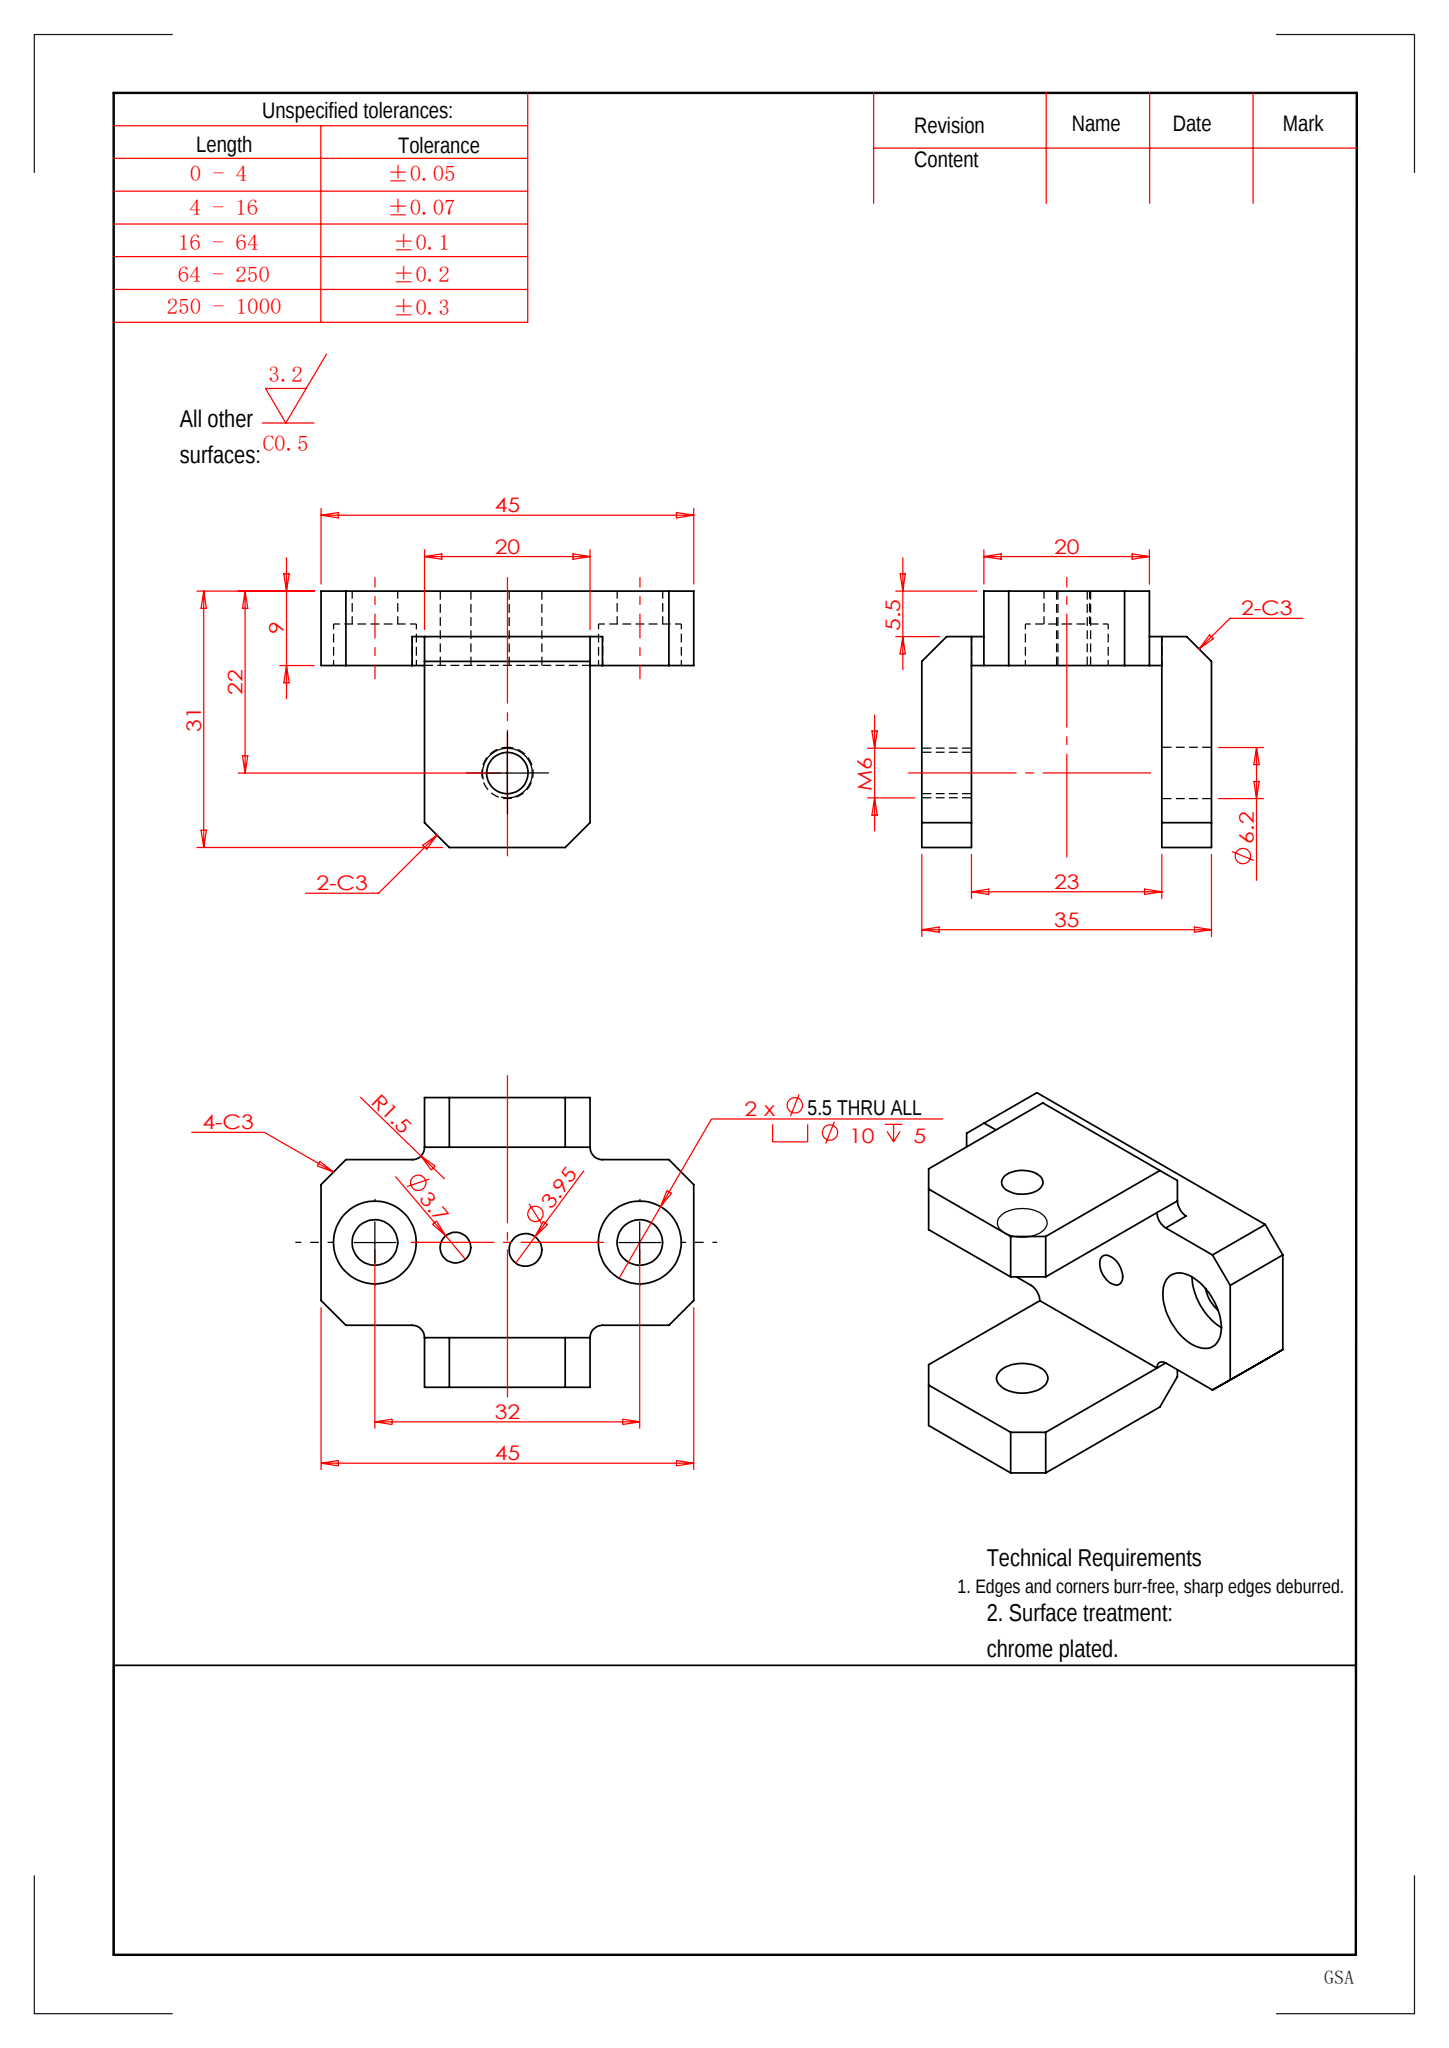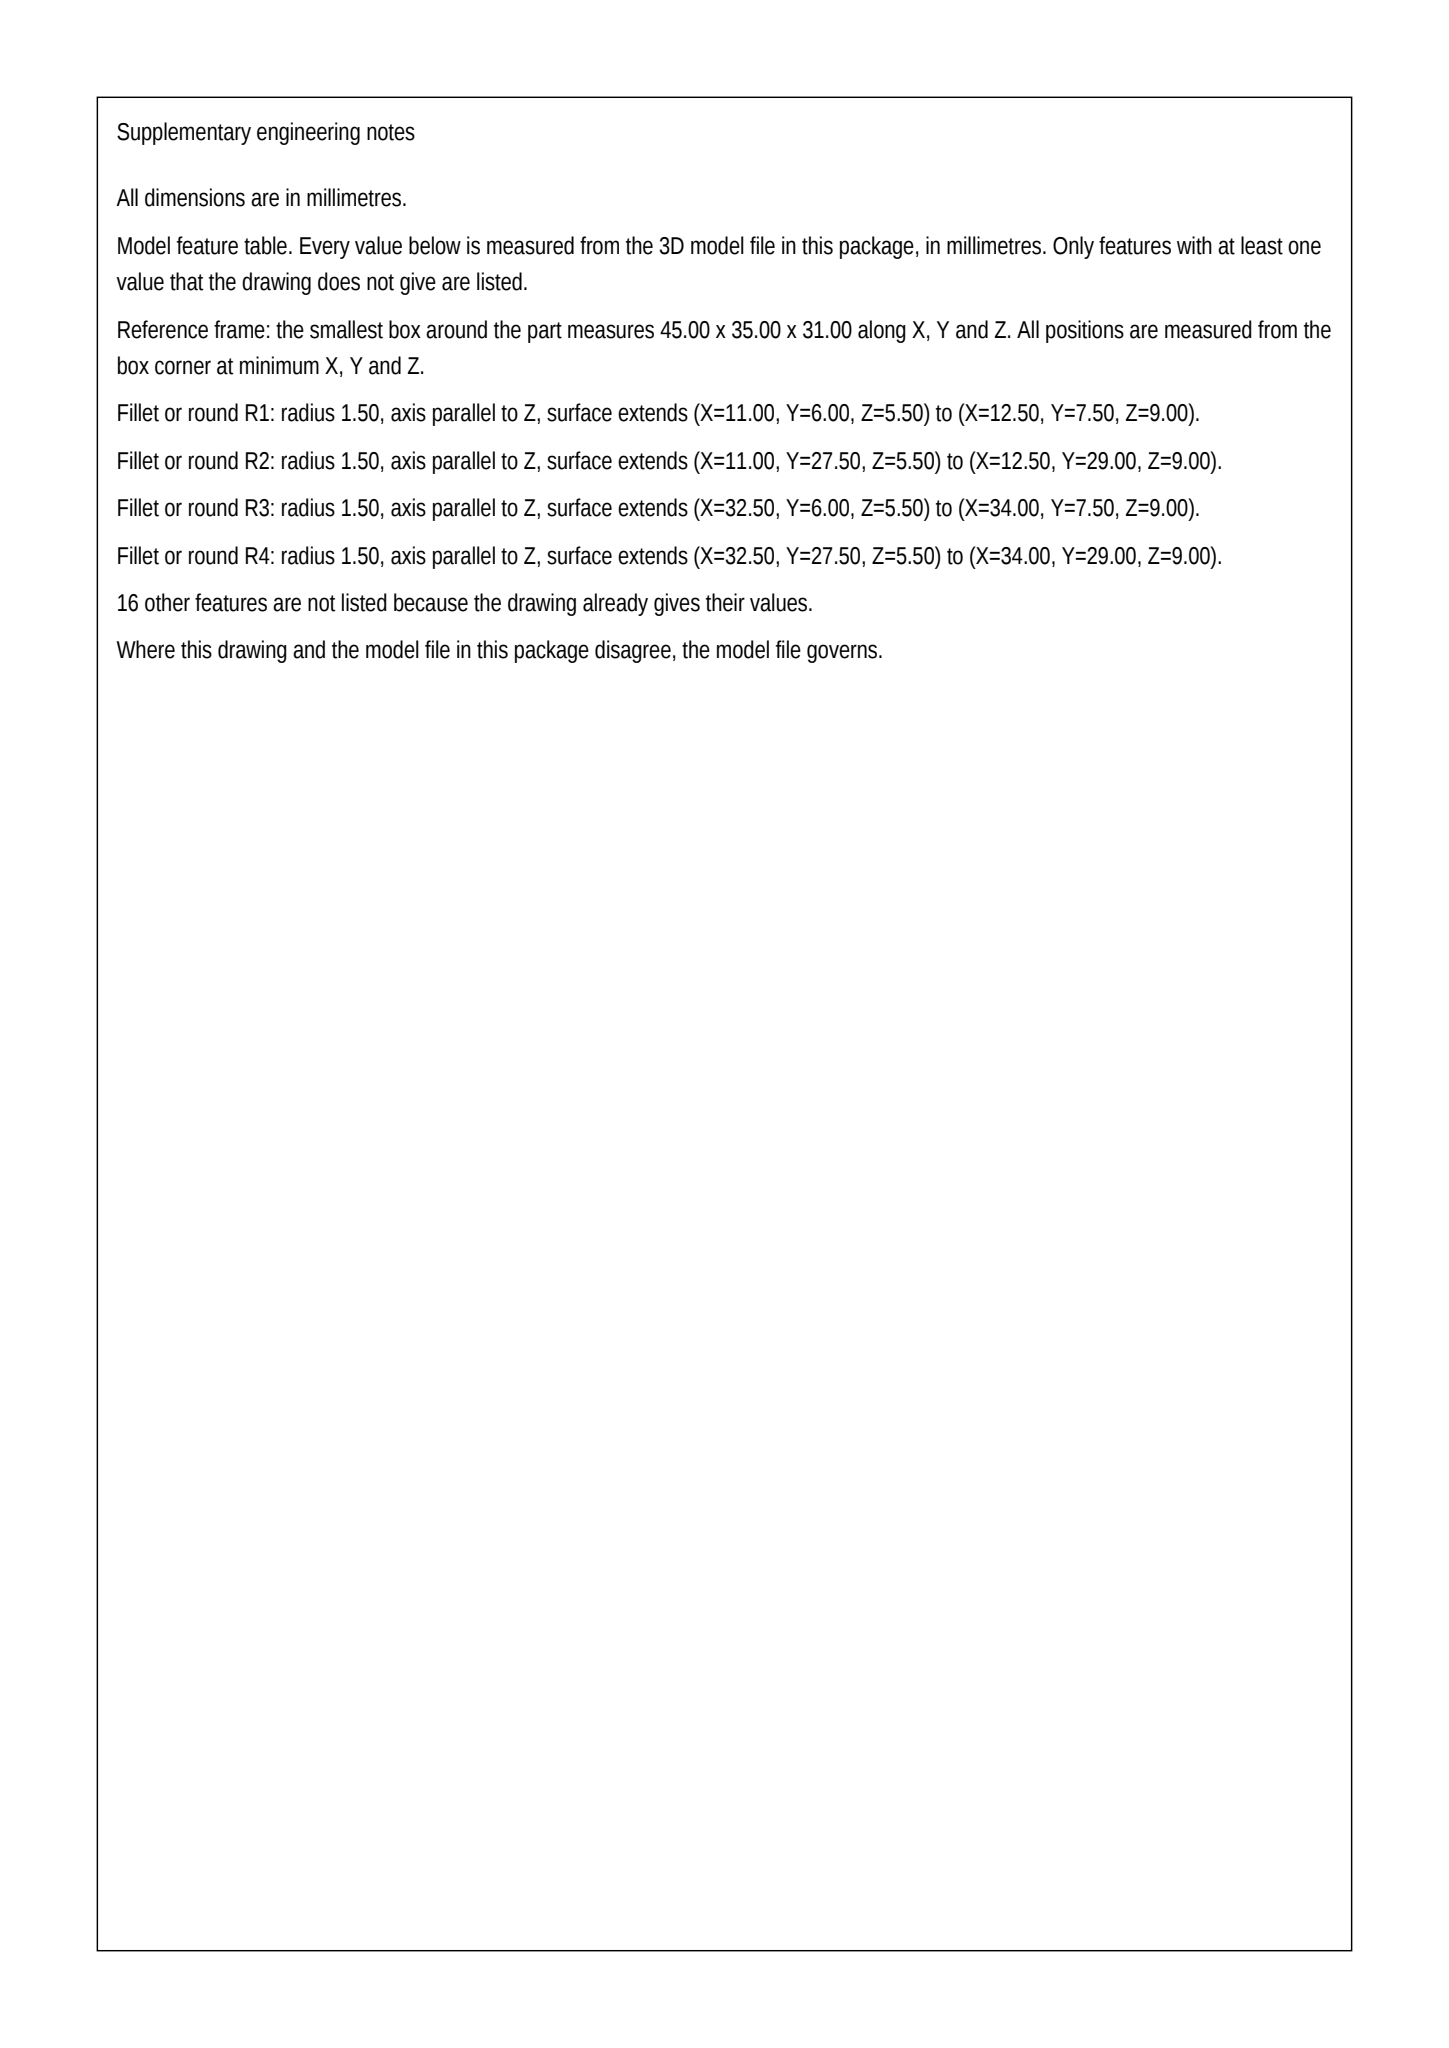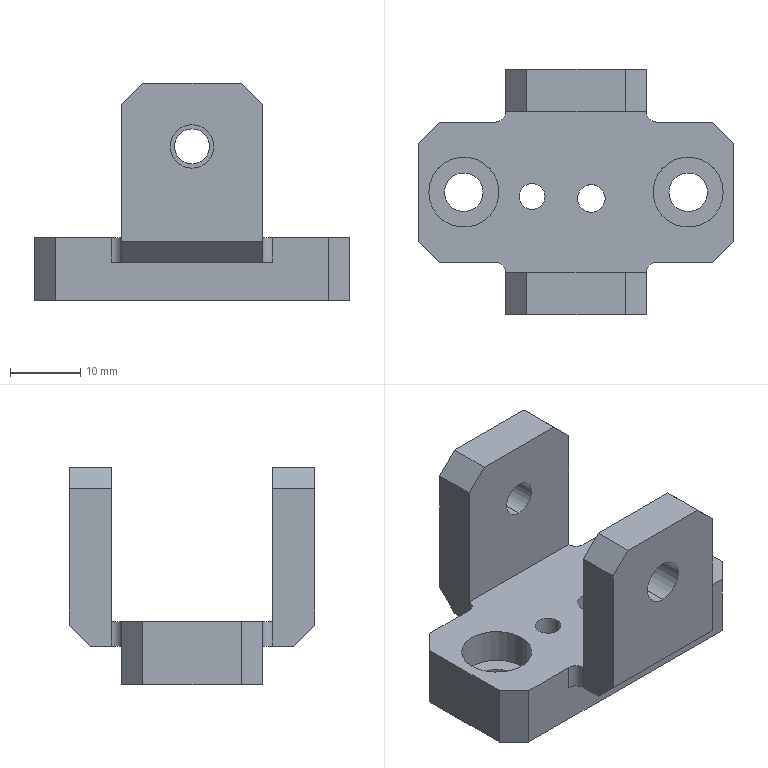Part | SolidWorks | mm | 1 solid | 50 faces | box 45 x 35 x 31 mm | volume 12505 mm3 | plane 30 | cylinder 20 | commonest cylinder face diameters 10 x4 5.5 x4 3 x4 3.949 x2 3.701 x2 5 x2 6.2 x2
build123d program:
from build123d import *

# Parameters (mm, degrees)
SKETCH1_W                                            = 45
SKETCH1_H                                            = 20
BOSS_EXTRUDE1_DEPTH                                  = 9
SKETCH2_W                                            = 20
SKETCH2_H                                            = 35
BOSS_EXTRUDE2_DEPTH                                  = 3.5
SKETCH3_W                                            = 20
SKETCH3_H                                            = 6
BOSS_EXTRUDE3_DEPTH                                  = 22
SKETCH4_R                                            = 3.1
CUT_EXTRUDE1_DEPTH                                   = 6
HOLE_SIZE_ACCORDING_TO_HEXAGON_SOCKET_HE_D           = 5.5
HOLE_SIZE_ACCORDING_TO_HEXAGON_SOCKET_HE_CBORE_D     = 10
HOLE_SIZE_ACCORDING_TO_HEXAGON_SOCKET_HE_CBORE_DEPTH = 5
M6_TAPPED_HOLE1_D                                    = 5
CHAMFER1_SIZE                                        = 3
FILLET1_R                                            = 1.5
SKETCH10_R                                           = 1.974
SKETCH10_R_2                                         = 1.85
CUT_EXTRUDE2_DEPTH                                   = 10


with BuildPart() as part:
    # Sketch1 → Boss-Extrude1 (new body)
    with BuildSketch(Plane.XY):
        Rectangle(SKETCH1_W, SKETCH1_H)
    extrude(amount=BOSS_EXTRUDE1_DEPTH)

    # Sketch2 → Boss-Extrude2 (add)
    with BuildSketch(Plane.XY.offset(9)):
        Rectangle(SKETCH2_W, SKETCH2_H)
    extrude(amount=-BOSS_EXTRUDE2_DEPTH)

    # Sketch3 → Boss-Extrude3 (add)
    with BuildSketch(Plane.XY.offset(9)):
        with Locations((0, 14.5)):
            Rectangle(SKETCH3_W, SKETCH3_H)
        with Locations((0, -14.5)):
            Rectangle(SKETCH3_W, SKETCH3_H)
    extrude(amount=BOSS_EXTRUDE3_DEPTH)

    # Sketch4 → Cut-Extrude1 (cut)
    with BuildSketch(Plane.XZ.offset(17.5)):
        with Locations(Location((0, 22, 0), (0, 0, 270))):
            Circle(SKETCH4_R)
    extrude(amount=-CUT_EXTRUDE1_DEPTH, mode=Mode.SUBTRACT)

    # Hole Size according to Hexagon Socket He (through all)
    with Locations(Plane.XY.offset(9)):
        with Locations((-16, 0), (16, 0)):
            CounterBoreHole(HOLE_SIZE_ACCORDING_TO_HEXAGON_SOCKET_HE_D / 2, HOLE_SIZE_ACCORDING_TO_HEXAGON_SOCKET_HE_CBORE_D / 2, HOLE_SIZE_ACCORDING_TO_HEXAGON_SOCKET_HE_CBORE_DEPTH)

    # M6 Tapped Hole1 (through all)
    with Locations(Plane(origin=(0, -17.5, 22), x_dir=(0, 0, -1), z_dir=(0, -1, 0))):
        with Locations((0, 0)):
            Hole(M6_TAPPED_HOLE1_D / 2)

    # Chamfer1
    chamfer1_edges = [part.edges().sort_by_distance(p)[0] for p in [
        (0, -17.5, 5.5),
        (0, 17.5, 5.5),
        (-22.5, -10, 4.5),
        (-22.5, 10, 4.5),
        (22.5, -10, 4.5),
        (22.5, 10, 4.5),
        (-10, 14.5, 31),
        (10, 14.5, 31),
        (-10, -14.5, 31),
        (10, -14.5, 31),
    ]]
    chamfer(chamfer1_edges, length=CHAMFER1_SIZE)

    # Fillet1
    fillet1_edges = [part.edges().sort_by_distance(p)[0] for p in [
        (-10, -10, 7.25),
        (10, -10, 7.25),
        (10, 10, 7.25),
        (-10, 10, 7.25),
    ]]
    fillet(fillet1_edges, radius=FILLET1_R)

    # Sketch10 → Cut-Extrude2 (cut)
    with BuildSketch(Plane.XY.offset(9)):
        with Locations((2.182, -0.9014)):
            Circle(SKETCH10_R)
        with Locations((-6.262, -0.6168)):
            Circle(SKETCH10_R_2)
    extrude(amount=-CUT_EXTRUDE2_DEPTH, mode=Mode.SUBTRACT)


solid = part.part